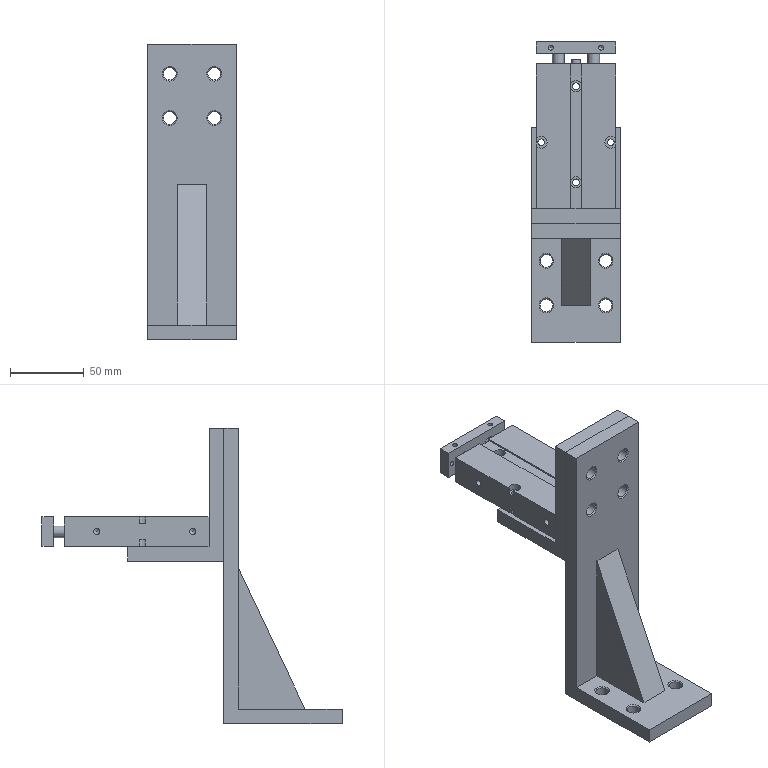Assembly | NX | mm | 6 component files | 12 solids | 275 faces | box 60 x 203 x 200 mm | volume 390831 mm3 | plane 129 | cone 74 | cylinder 64 | torus 8 | commonest cylinder face diameters 8.5 x12 8 x8 10 x6 3.3 x6 6 x5 5.795 x4 4.5 x4 7.5 x4
Bill of materials:
unnamed part 1 | 1 |  | Bracket with a tall rectangular upright plate. A rectangular base flange sits at the bottom, a thinner flange sticks out the opposite way partway up, and a sloped triangular gusset joins the upright to the base.
GB-T70.1-2000,M6x16 | 4 |  | Hexagon Socket Head Cap Screw, GB-T 70.1-2000,M6x16
unnamed part 2 | 1 |  | Rectangular block body with a separate end plate set a short distance away. Two parallel cylindrical rods and a smaller central stub join the plate to the body. Overall it looks like a compact guided-rod linear unit, but this is not confirmed.
Mates:
1. touch align | dual_axis_cylinder 1 face | assembly face
2. distance | dual_axis_cylinder 1 face | assembly face
3. touch align | dual_axis_cylinder 1 edge | assembly face
4. concentric | GB-T70_1-2000_M6x16 4 edge | assembly edge
5. concentric | GB-T70_1-2000_M6x16 3 edge | assembly edge
6. concentric | GB-T70_1-2000_M6x16 2 edge | assembly edge
7. concentric | GB-T70_1-2000_M6x16 1 edge | assembly edge